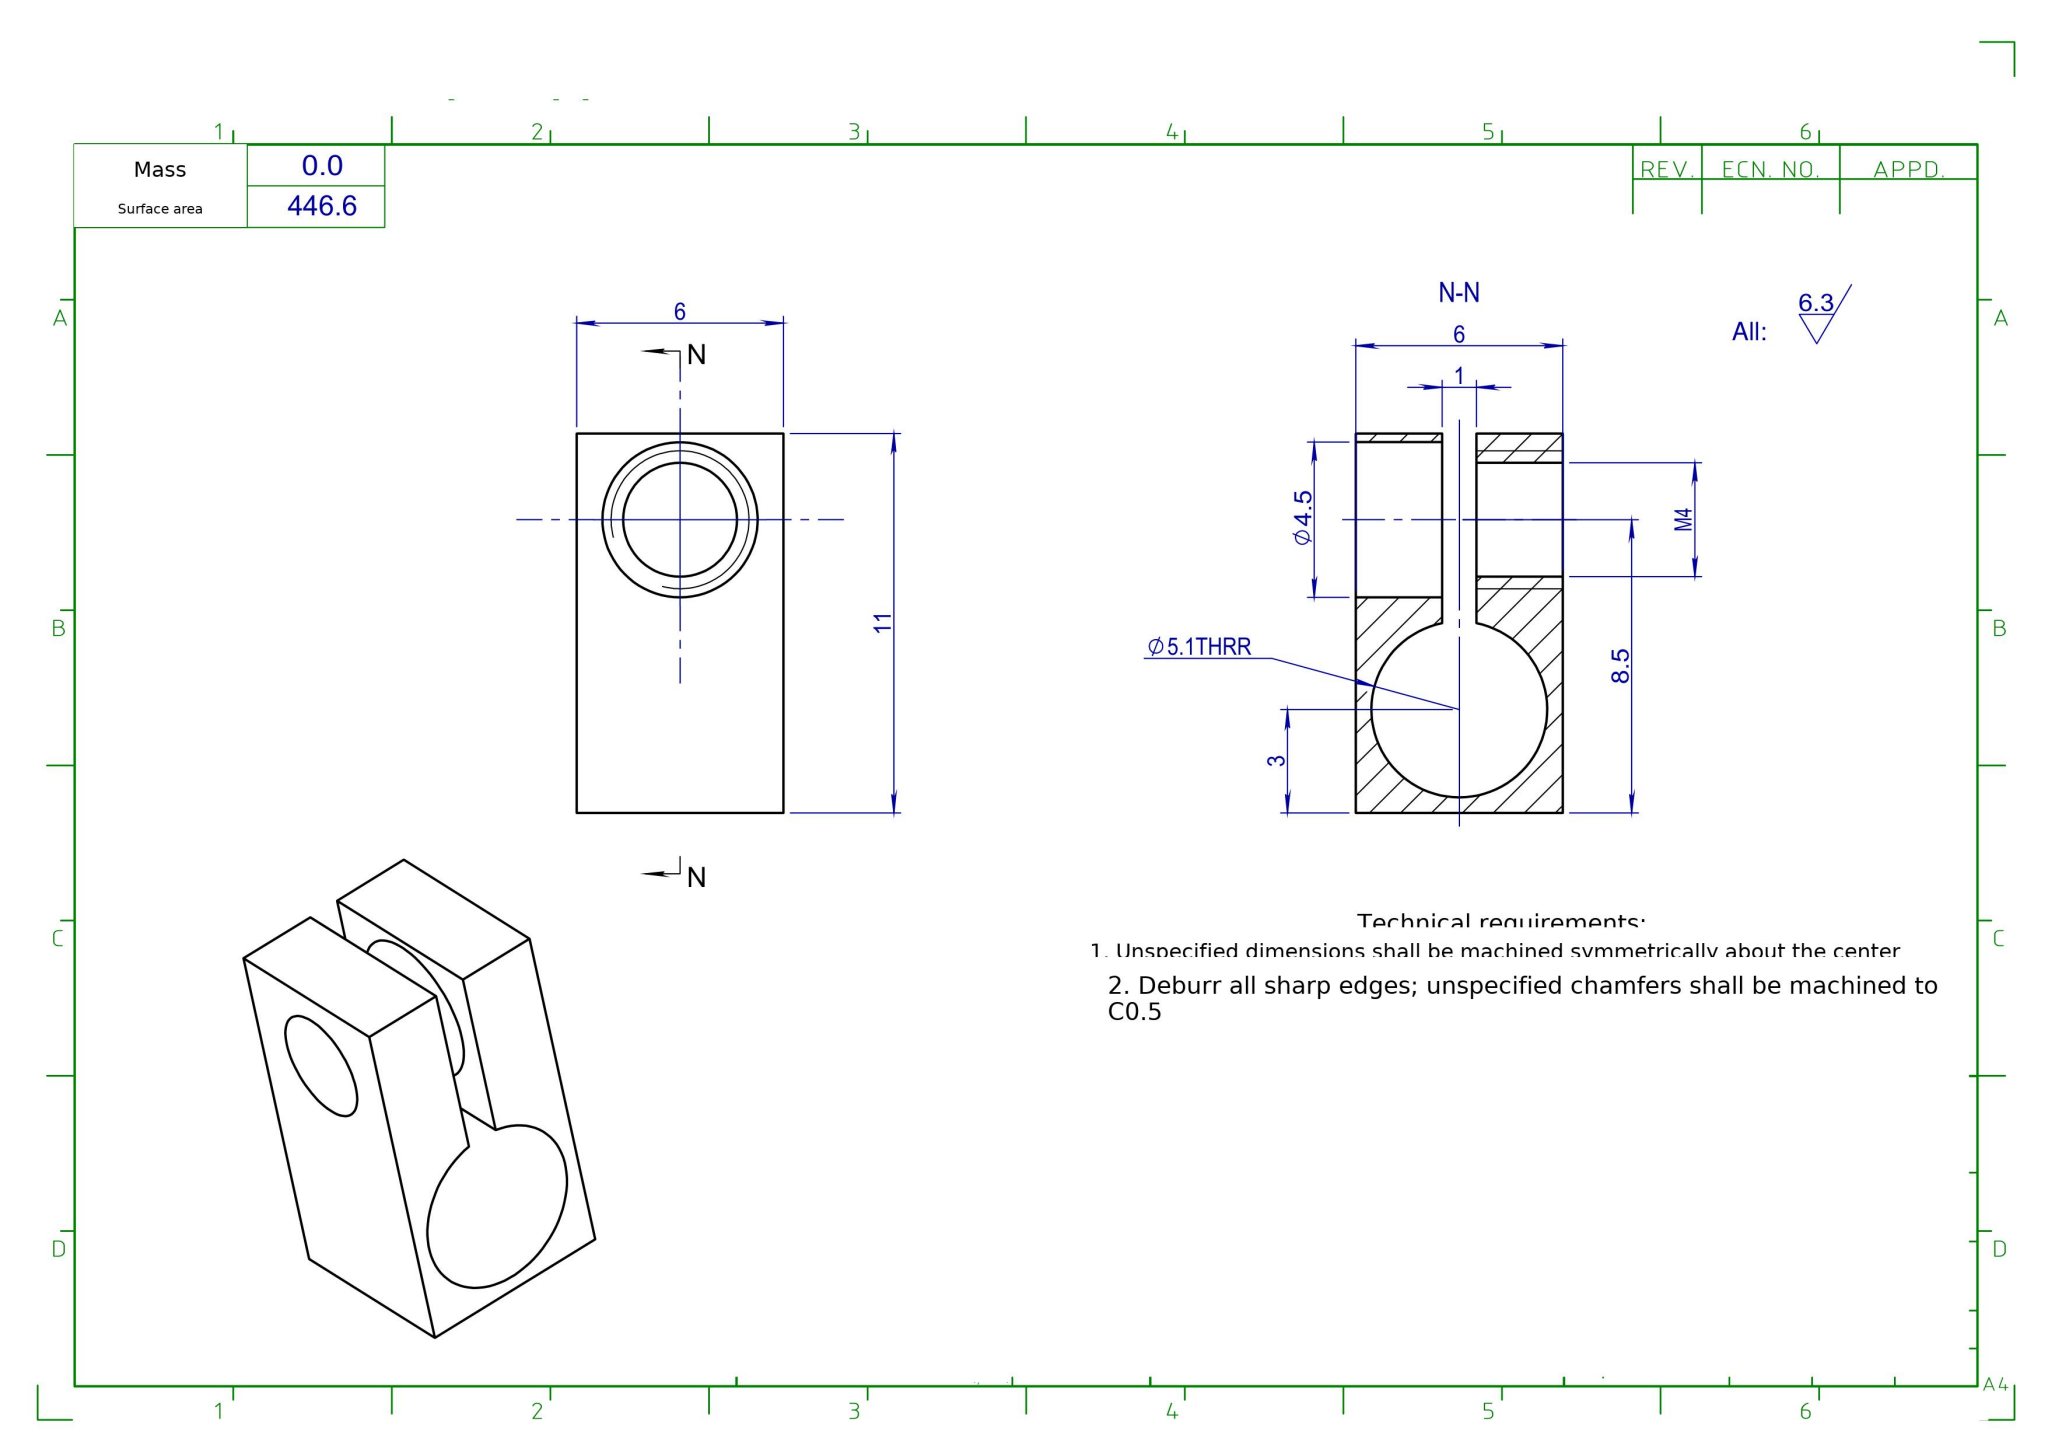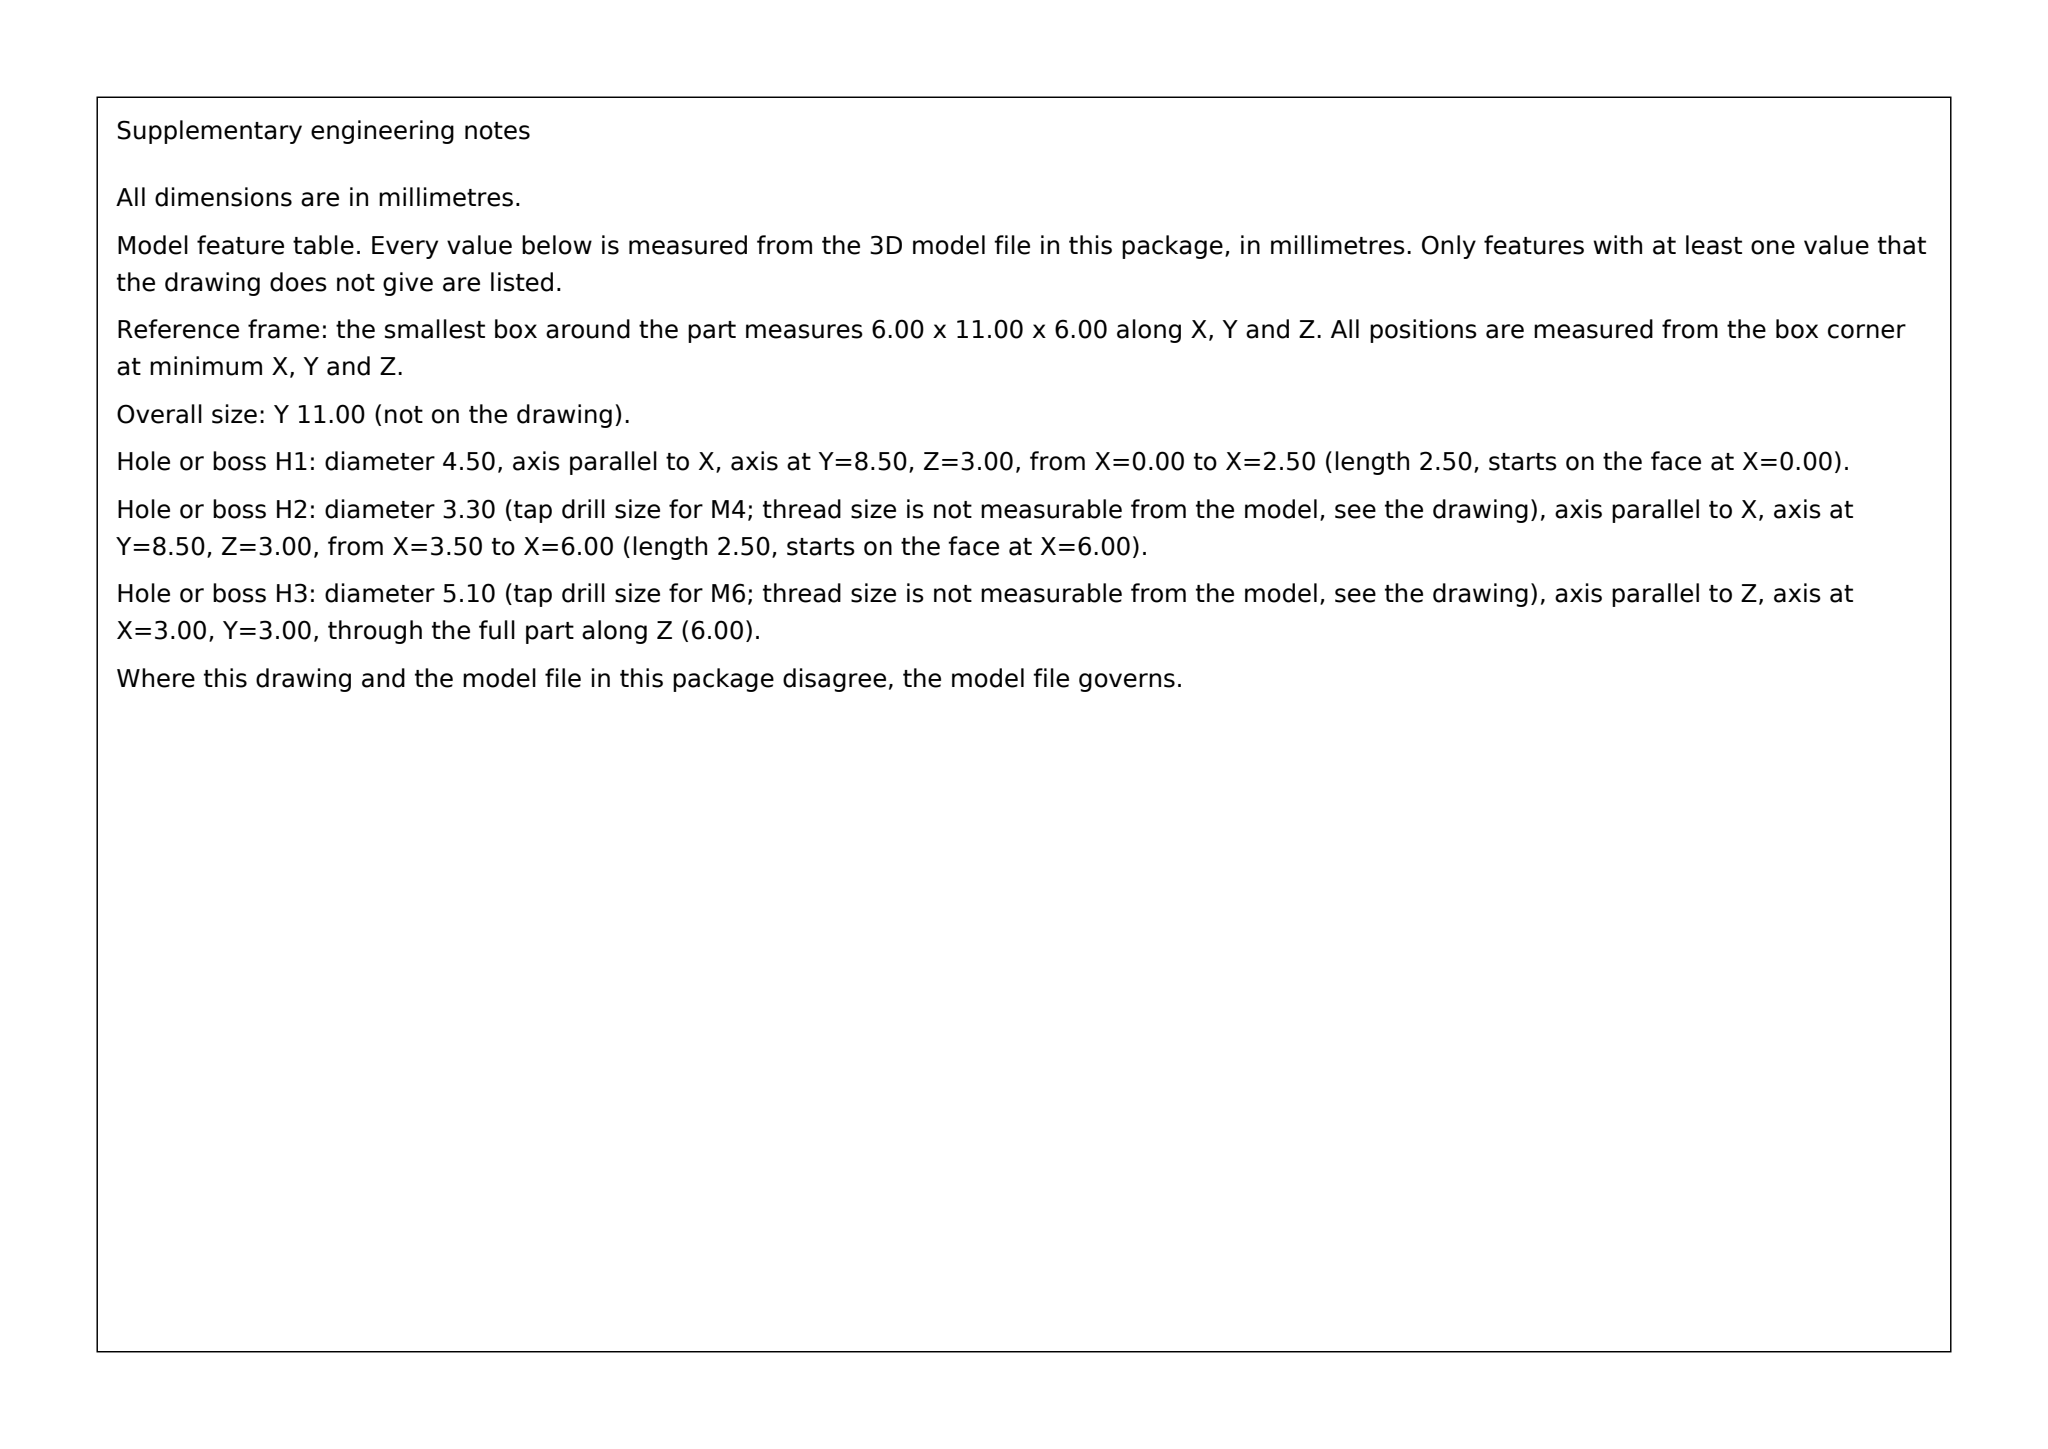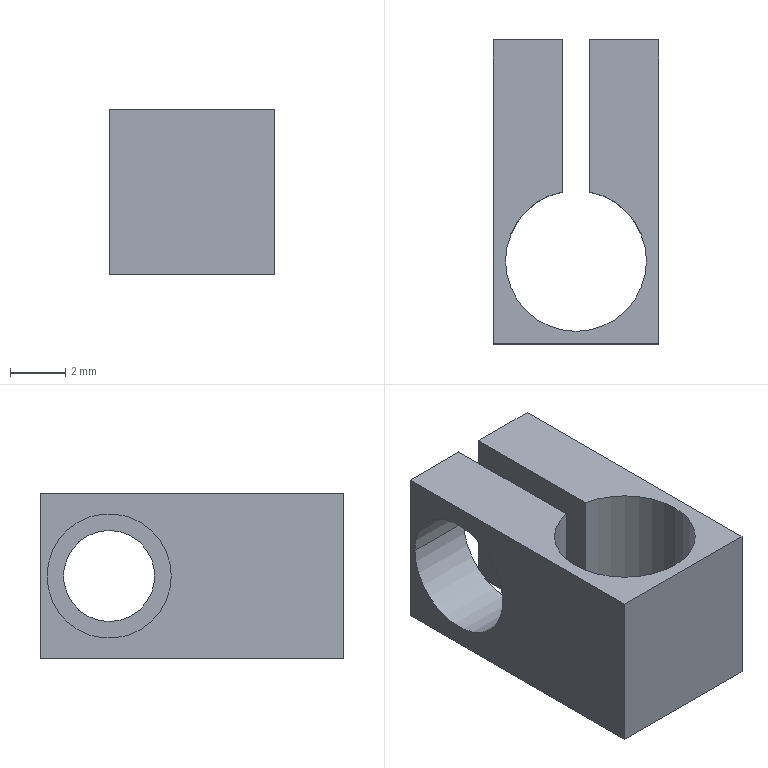Part | SolidWorks | mm | 1 solid | 16 faces | box 6 x 11 x 6 mm | volume 179 mm3 | plane 9 | cylinder 7 | commonest cylinder face diameters 5.1 x3 3.3 x2 4.5 x2
build123d program:
from build123d import *

# Parameters (mm, degrees)
SKETCH1_W             = 6
SKETCH1_H             = 11
EXTRUDE1_DEPTH        = 6
SKETCH2_R             = 2.55
CUT_EXTRUDE1_DEPTH    = 32.386
SKETCH4_W             = 1
SKETCH4_H             = 8
CUT_EXTRUDE3_DEPTH    = 32.386
SKETCH6_R             = 2.25
CUT_EXTRUDE5_DEPTH    = 2.5
M4_TAPPED_HOLE1_D     = 3.3
M4_TAPPED_HOLE1_DEPTH = 10.1
M4_TAPPED_HOLE1_TIP   = 0.9914


with BuildPart() as part:
    # Sketch1 → Extrude1 (new body)
    with BuildSketch(Plane.XY):
        with Locations((-13.52, -20.503)):
            Rectangle(SKETCH1_W, SKETCH1_H)
    extrude(amount=EXTRUDE1_DEPTH)

    # Sketch2 → Cut-Extrude1 (cut, through all)
    with BuildSketch(Plane.XY.offset(6)):
        with Locations((-13.52, -23.003)):
            Circle(SKETCH2_R)
    extrude(amount=-CUT_EXTRUDE1_DEPTH, mode=Mode.SUBTRACT)

    # Sketch4 → Cut-Extrude3 (cut, through all)
    with BuildSketch(Plane.XY.offset(6)):
        with Locations((-13.52, -19.003)):
            Rectangle(SKETCH4_W, SKETCH4_H)
    extrude(amount=-CUT_EXTRUDE3_DEPTH, mode=Mode.SUBTRACT)

    # Sketch6 → Cut-Extrude5 (cut)
    with BuildSketch(Plane.ZY.offset(16.52)):
        with Locations(Location((3, -17.503, 0), (0, 0, 270))):
            Circle(SKETCH6_R)
    extrude(amount=-CUT_EXTRUDE5_DEPTH, mode=Mode.SUBTRACT)

    # M4 Tapped Hole1
    with Locations(Plane.ZY.offset(13.02)):
        with Locations((3, -17.503)):
            Hole(M4_TAPPED_HOLE1_D / 2, depth=M4_TAPPED_HOLE1_DEPTH)
            with Locations((0, 0, -(M4_TAPPED_HOLE1_DEPTH + M4_TAPPED_HOLE1_TIP / 2))):  # 118° drill point
                Cone(0, M4_TAPPED_HOLE1_D / 2, M4_TAPPED_HOLE1_TIP, mode=Mode.SUBTRACT)


solid = part.part
STEP:
#1=CARTESIAN_POINT('',(-10.52,-17.503,1.35));
#2=VERTEX_POINT('',#1);
#3=CARTESIAN_POINT('',(-10.52,-17.503,4.65));
#4=VERTEX_POINT('',#3);
#5=CARTESIAN_POINT('',(-10.52,-17.503,3.));
#6=DIRECTION('',(-1.,-0.,0.));
#7=DIRECTION('',(0.,-1.,0.));
#8=AXIS2_PLACEMENT_3D('',#5,#6,#7);
#9=CIRCLE('',#8,1.65);
#10=EDGE_CURVE('',#2,#4,#9,.T.);
#11=ORIENTED_EDGE('',*,*,#10,.F.);
#12=CARTESIAN_POINT('',(-13.02,-17.503,1.35));
#13=VERTEX_POINT('',#12);
#14=CARTESIAN_POINT('',(-13.02,-17.503,1.35));
#15=DIRECTION('',(-1.,0.,0.));
#16=VECTOR('',#15,1000.);
#17=LINE('',#14,#16);
#18=EDGE_CURVE('',#2,#13,#17,.T.);
#19=ORIENTED_EDGE('',*,*,#18,.T.);
#20=CARTESIAN_POINT('',(-13.02,-17.503,4.65));
#21=VERTEX_POINT('',#20);
#22=CARTESIAN_POINT('',(-13.02,-17.503,3.));
#23=DIRECTION('',(-1.,0.,0.));
#24=DIRECTION('',(0.,0.,1.));
#25=AXIS2_PLACEMENT_3D('',#22,#23,#24);
#26=CIRCLE('',#25,1.65);
#27=EDGE_CURVE('',#13,#21,#26,.T.);
#28=ORIENTED_EDGE('',*,*,#27,.T.);
#29=CARTESIAN_POINT('',(-13.02,-17.503,4.65));
#30=DIRECTION('',(-1.,0.,0.));
#31=VECTOR('',#30,1000.);
#32=LINE('',#29,#31);
#33=EDGE_CURVE('',#4,#21,#32,.T.);
#34=ORIENTED_EDGE('',*,*,#33,.F.);
#35=EDGE_LOOP('',(#11,#19,#28,#34));
#36=FACE_OUTER_BOUND('',#35,.T.);
#37=CARTESIAN_POINT('',(-13.02,-17.503,3.));
#38=DIRECTION('',(-1.,0.,0.));
#39=DIRECTION('',(0.,0.,1.));
#40=AXIS2_PLACEMENT_3D('',#37,#38,#39);
#41=CYLINDRICAL_SURFACE('',#40,1.65);
#42=ADVANCED_FACE('',(#36),#41,.F.);
#43=CARTESIAN_POINT('',(-14.02,-15.253,3.));
#44=VERTEX_POINT('',#43);
#45=CARTESIAN_POINT('',(-14.02,-19.753,3.));
#46=VERTEX_POINT('',#45);
#47=CARTESIAN_POINT('',(-14.02,-17.503,3.));
#48=DIRECTION('',(-1.,-0.,0.));
#49=DIRECTION('',(0.,-1.,0.));
#50=AXIS2_PLACEMENT_3D('',#47,#48,#49);
#51=CIRCLE('',#50,2.25);
#52=EDGE_CURVE('',#44,#46,#51,.T.);
#53=ORIENTED_EDGE('',*,*,#52,.F.);
#54=CARTESIAN_POINT('',(-16.52,-15.253,3.));
#55=VERTEX_POINT('',#54);
#56=CARTESIAN_POINT('',(-14.02,-15.253,3.));
#57=DIRECTION('',(-1.,-0.,0.));
#58=VECTOR('',#57,1000.);
#59=LINE('',#56,#58);
#60=EDGE_CURVE('',#44,#55,#59,.T.);
#61=ORIENTED_EDGE('',*,*,#60,.T.);
#62=CARTESIAN_POINT('',(-16.52,-19.753,3.));
#63=VERTEX_POINT('',#62);
#64=CARTESIAN_POINT('',(-16.52,-17.503,3.));
#65=DIRECTION('',(-1.,-0.,0.));
#66=DIRECTION('',(0.,-1.,0.));
#67=AXIS2_PLACEMENT_3D('',#64,#65,#66);
#68=CIRCLE('',#67,2.25);
#69=EDGE_CURVE('',#55,#63,#68,.T.);
#70=ORIENTED_EDGE('',*,*,#69,.T.);
#71=CARTESIAN_POINT('',(-14.02,-19.753,3.));
#72=DIRECTION('',(-1.,-0.,0.));
#73=VECTOR('',#72,1000.);
#74=LINE('',#71,#73);
#75=EDGE_CURVE('',#46,#63,#74,.T.);
#76=ORIENTED_EDGE('',*,*,#75,.F.);
#77=EDGE_LOOP('',(#53,#61,#70,#76));
#78=FACE_OUTER_BOUND('',#77,.T.);
#79=CARTESIAN_POINT('',(-14.02,-17.503,3.));
#80=DIRECTION('',(-1.,-0.,0.));
#81=DIRECTION('',(0.,-1.,0.));
#82=AXIS2_PLACEMENT_3D('',#79,#80,#81);
#83=CYLINDRICAL_SURFACE('',#82,2.25);
#84=ADVANCED_FACE('',(#78),#83,.F.);
#85=CARTESIAN_POINT('',(-16.07,-23.003,0.));
#86=VERTEX_POINT('',#85);
#87=CARTESIAN_POINT('',(-10.97,-23.003,0.));
#88=VERTEX_POINT('',#87);
#89=CARTESIAN_POINT('',(-13.52,-23.003,0.));
#90=DIRECTION('',(0.,0.,1.));
#91=DIRECTION('',(1.,0.,0.));
#92=AXIS2_PLACEMENT_3D('',#89,#90,#91);
#93=CIRCLE('',#92,2.55);
#94=EDGE_CURVE('',#86,#88,#93,.T.);
#95=ORIENTED_EDGE('',*,*,#94,.F.);
#96=CARTESIAN_POINT('',(-16.07,-23.003,6.));
#97=VERTEX_POINT('',#96);
#98=CARTESIAN_POINT('',(-16.07,-23.003,0.));
#99=DIRECTION('',(0.,0.,1.));
#100=VECTOR('',#99,1000.);
#101=LINE('',#98,#100);
#102=EDGE_CURVE('',#86,#97,#101,.T.);
#103=ORIENTED_EDGE('',*,*,#102,.T.);
#104=CARTESIAN_POINT('',(-10.97,-23.003,6.));
#105=VERTEX_POINT('',#104);
#106=CARTESIAN_POINT('',(-13.52,-23.003,6.));
#107=DIRECTION('',(0.,0.,1.));
#108=DIRECTION('',(1.,0.,0.));
#109=AXIS2_PLACEMENT_3D('',#106,#107,#108);
#110=CIRCLE('',#109,2.55);
#111=EDGE_CURVE('',#97,#105,#110,.T.);
#112=ORIENTED_EDGE('',*,*,#111,.T.);
#113=CARTESIAN_POINT('',(-10.97,-23.003,0.));
#114=DIRECTION('',(0.,0.,1.));
#115=VECTOR('',#114,1000.);
#116=LINE('',#113,#115);
#117=EDGE_CURVE('',#88,#105,#116,.T.);
#118=ORIENTED_EDGE('',*,*,#117,.F.);
#119=EDGE_LOOP('',(#95,#103,#112,#118));
#120=FACE_OUTER_BOUND('',#119,.T.);
#121=CARTESIAN_POINT('',(-13.52,-23.003,0.));
#122=DIRECTION('',(0.,0.,1.));
#123=DIRECTION('',(1.,0.,0.));
#124=AXIS2_PLACEMENT_3D('',#121,#122,#123);
#125=CYLINDRICAL_SURFACE('',#124,2.55);
#126=ADVANCED_FACE('',(#120),#125,.F.);
#127=CARTESIAN_POINT('',(-13.02,-20.502,0.));
#128=VERTEX_POINT('',#127);
#129=CARTESIAN_POINT('',(-13.52,-23.003,0.));
#130=DIRECTION('',(0.,0.,1.));
#131=DIRECTION('',(1.,0.,0.));
#132=AXIS2_PLACEMENT_3D('',#129,#130,#131);
#133=CIRCLE('',#132,2.55);
#134=EDGE_CURVE('',#88,#128,#133,.T.);
#135=ORIENTED_EDGE('',*,*,#134,.F.);
#136=ORIENTED_EDGE('',*,*,#117,.T.);
#137=CARTESIAN_POINT('',(-13.02,-20.502,6.));
#138=VERTEX_POINT('',#137);
#139=CARTESIAN_POINT('',(-13.52,-23.003,6.));
#140=DIRECTION('',(0.,0.,1.));
#141=DIRECTION('',(1.,0.,0.));
#142=AXIS2_PLACEMENT_3D('',#139,#140,#141);
#143=CIRCLE('',#142,2.55);
#144=EDGE_CURVE('',#105,#138,#143,.T.);
#145=ORIENTED_EDGE('',*,*,#144,.T.);
#146=CARTESIAN_POINT('',(-13.02,-20.502,0.));
#147=DIRECTION('',(0.,0.,-1.));
#148=VECTOR('',#147,1000.);
#149=LINE('',#146,#148);
#150=EDGE_CURVE('',#138,#128,#149,.T.);
#151=ORIENTED_EDGE('',*,*,#150,.T.);
#152=EDGE_LOOP('',(#135,#136,#145,#151));
#153=FACE_OUTER_BOUND('',#152,.T.);
#154=CARTESIAN_POINT('',(-13.52,-23.003,0.));
#155=DIRECTION('',(0.,0.,1.));
#156=DIRECTION('',(1.,0.,0.));
#157=AXIS2_PLACEMENT_3D('',#154,#155,#156);
#158=CYLINDRICAL_SURFACE('',#157,2.55);
#159=ADVANCED_FACE('',(#153),#158,.F.);
#160=CARTESIAN_POINT('',(-14.02,-15.003,6.));
#161=VERTEX_POINT('',#160);
#162=CARTESIAN_POINT('',(-16.52,-15.003,6.));
#163=VERTEX_POINT('',#162);
#164=CARTESIAN_POINT('',(-16.52,-15.003,6.));
#165=DIRECTION('',(-1.,0.,0.));
#166=VECTOR('',#165,1000.);
#167=LINE('',#164,#166);
#168=EDGE_CURVE('',#161,#163,#167,.T.);
#169=ORIENTED_EDGE('',*,*,#168,.F.);
#170=CARTESIAN_POINT('',(-14.02,-15.003,0.));
#171=VERTEX_POINT('',#170);
#172=CARTESIAN_POINT('',(-14.02,-15.003,0.));
#173=DIRECTION('',(0.,0.,1.));
#174=VECTOR('',#173,1000.);
#175=LINE('',#172,#174);
#176=EDGE_CURVE('',#171,#161,#175,.T.);
#177=ORIENTED_EDGE('',*,*,#176,.F.);
#178=CARTESIAN_POINT('',(-16.52,-15.003,0.));
#179=VERTEX_POINT('',#178);
#180=CARTESIAN_POINT('',(-16.52,-15.003,0.));
#181=DIRECTION('',(-1.,0.,0.));
#182=VECTOR('',#181,1000.);
#183=LINE('',#180,#182);
#184=EDGE_CURVE('',#171,#179,#183,.T.);
#185=ORIENTED_EDGE('',*,*,#184,.T.);
#186=CARTESIAN_POINT('',(-16.52,-15.003,6.));
#187=DIRECTION('',(0.,0.,-1.));
#188=VECTOR('',#187,1000.);
#189=LINE('',#186,#188);
#190=EDGE_CURVE('',#163,#179,#189,.T.);
#191=ORIENTED_EDGE('',*,*,#190,.F.);
#192=EDGE_LOOP('',(#169,#177,#185,#191));
#193=FACE_OUTER_BOUND('',#192,.T.);
#194=CARTESIAN_POINT('',(-16.52,-15.003,6.));
#195=DIRECTION('',(0.,-1.,0.));
#196=DIRECTION('',(0.,0.,-1.));
#197=AXIS2_PLACEMENT_3D('',#194,#195,#196);
#198=PLANE('',#197);
#199=ADVANCED_FACE('',(#193),#198,.F.);
#200=CARTESIAN_POINT('',(-16.52,-17.503,3.));
#201=DIRECTION('',(-1.,-0.,0.));
#202=DIRECTION('',(0.,-1.,0.));
#203=AXIS2_PLACEMENT_3D('',#200,#201,#202);
#204=CIRCLE('',#203,2.25);
#205=EDGE_CURVE('',#63,#55,#204,.T.);
#206=ORIENTED_EDGE('',*,*,#205,.F.);
#207=ORIENTED_EDGE('',*,*,#69,.F.);
#208=EDGE_LOOP('',(#206,#207));
#209=FACE_BOUND('',#208,.T.);
#210=CARTESIAN_POINT('',(-16.52,-26.003,0.));
#211=VERTEX_POINT('',#210);
#212=CARTESIAN_POINT('',(-16.52,-15.003,0.));
#213=DIRECTION('',(0.,-1.,0.));
#214=VECTOR('',#213,1000.);
#215=LINE('',#212,#214);
#216=EDGE_CURVE('',#179,#211,#215,.T.);
#217=ORIENTED_EDGE('',*,*,#216,.T.);
#218=CARTESIAN_POINT('',(-16.52,-26.003,6.));
#219=VERTEX_POINT('',#218);
#220=CARTESIAN_POINT('',(-16.52,-26.003,6.));
#221=DIRECTION('',(0.,0.,-1.));
#222=VECTOR('',#221,1000.);
#223=LINE('',#220,#222);
#224=EDGE_CURVE('',#219,#211,#223,.T.);
#225=ORIENTED_EDGE('',*,*,#224,.F.);
#226=CARTESIAN_POINT('',(-16.52,-15.003,6.));
#227=DIRECTION('',(0.,-1.,0.));
#228=VECTOR('',#227,1000.);
#229=LINE('',#226,#228);
#230=EDGE_CURVE('',#163,#219,#229,.T.);
#231=ORIENTED_EDGE('',*,*,#230,.F.);
#232=ORIENTED_EDGE('',*,*,#190,.T.);
#233=EDGE_LOOP('',(#217,#225,#231,#232));
#234=FACE_OUTER_BOUND('',#233,.T.);
#235=CARTESIAN_POINT('',(-16.52,-15.003,6.));
#236=DIRECTION('',(1.,0.,0.));
#237=DIRECTION('',(0.,0.,-1.));
#238=AXIS2_PLACEMENT_3D('',#235,#236,#237);
#239=PLANE('',#238);
#240=ADVANCED_FACE('',(#209,#234),#239,.F.);
#241=CARTESIAN_POINT('',(-10.52,-26.003,0.));
#242=VERTEX_POINT('',#241);
#243=CARTESIAN_POINT('',(-16.52,-26.003,0.));
#244=DIRECTION('',(1.,0.,0.));
#245=VECTOR('',#244,1000.);
#246=LINE('',#243,#245);
#247=EDGE_CURVE('',#211,#242,#246,.T.);
#248=ORIENTED_EDGE('',*,*,#247,.T.);
#249=CARTESIAN_POINT('',(-10.52,-26.003,6.));
#250=VERTEX_POINT('',#249);
#251=CARTESIAN_POINT('',(-10.52,-26.003,6.));
#252=DIRECTION('',(0.,0.,-1.));
#253=VECTOR('',#252,1000.);
#254=LINE('',#251,#253);
#255=EDGE_CURVE('',#250,#242,#254,.T.);
#256=ORIENTED_EDGE('',*,*,#255,.F.);
#257=CARTESIAN_POINT('',(-16.52,-26.003,6.));
#258=DIRECTION('',(1.,0.,0.));
#259=VECTOR('',#258,1000.);
#260=LINE('',#257,#259);
#261=EDGE_CURVE('',#219,#250,#260,.T.);
#262=ORIENTED_EDGE('',*,*,#261,.F.);
#263=ORIENTED_EDGE('',*,*,#224,.T.);
#264=EDGE_LOOP('',(#248,#256,#262,#263));
#265=FACE_OUTER_BOUND('',#264,.T.);
#266=CARTESIAN_POINT('',(-16.52,-26.003,6.));
#267=DIRECTION('',(0.,1.,0.));
#268=DIRECTION('',(0.,0.,1.));
#269=AXIS2_PLACEMENT_3D('',#266,#267,#268);
#270=PLANE('',#269);
#271=ADVANCED_FACE('',(#265),#270,.F.);
#272=CARTESIAN_POINT('',(-10.52,-17.503,3.));
#273=DIRECTION('',(-1.,-0.,0.));
#274=DIRECTION('',(0.,-1.,0.));
#275=AXIS2_PLACEMENT_3D('',#272,#273,#274);
#276=CIRCLE('',#275,1.65);
#277=EDGE_CURVE('',#4,#2,#276,.T.);
#278=ORIENTED_EDGE('',*,*,#277,.T.);
#279=ORIENTED_EDGE('',*,*,#10,.T.);
#280=EDGE_LOOP('',(#278,#279));
#281=FACE_BOUND('',#280,.T.);
#282=CARTESIAN_POINT('',(-10.52,-15.003,0.));
#283=VERTEX_POINT('',#282);
#284=CARTESIAN_POINT('',(-10.52,-15.003,0.));
#285=DIRECTION('',(-0.,1.,0.));
#286=VECTOR('',#285,1000.);
#287=LINE('',#284,#286);
#288=EDGE_CURVE('',#242,#283,#287,.T.);
#289=ORIENTED_EDGE('',*,*,#288,.T.);
#290=CARTESIAN_POINT('',(-10.52,-15.003,6.));
#291=VERTEX_POINT('',#290);
#292=CARTESIAN_POINT('',(-10.52,-15.003,6.));
#293=DIRECTION('',(0.,0.,-1.));
#294=VECTOR('',#293,1000.);
#295=LINE('',#292,#294);
#296=EDGE_CURVE('',#291,#283,#295,.T.);
#297=ORIENTED_EDGE('',*,*,#296,.F.);
#298=CARTESIAN_POINT('',(-10.52,-15.003,6.));
#299=DIRECTION('',(-0.,1.,0.));
#300=VECTOR('',#299,1000.);
#301=LINE('',#298,#300);
#302=EDGE_CURVE('',#250,#291,#301,.T.);
#303=ORIENTED_EDGE('',*,*,#302,.F.);
#304=ORIENTED_EDGE('',*,*,#255,.T.);
#305=EDGE_LOOP('',(#289,#297,#303,#304));
#306=FACE_OUTER_BOUND('',#305,.T.);
#307=CARTESIAN_POINT('',(-10.52,-15.003,6.));
#308=DIRECTION('',(-1.,-0.,0.));
#309=DIRECTION('',(0.,-1.,0.));
#310=AXIS2_PLACEMENT_3D('',#307,#308,#309);
#311=PLANE('',#310);
#312=ADVANCED_FACE('',(#281,#306),#311,.F.);
#313=CARTESIAN_POINT('',(-13.02,-15.003,0.));
#314=VERTEX_POINT('',#313);
#315=CARTESIAN_POINT('',(-16.52,-15.003,0.));
#316=DIRECTION('',(-1.,0.,0.));
#317=VECTOR('',#316,1000.);
#318=LINE('',#315,#317);
#319=EDGE_CURVE('',#283,#314,#318,.T.);
#320=ORIENTED_EDGE('',*,*,#319,.T.);
#321=CARTESIAN_POINT('',(-13.02,-15.003,6.));
#322=VERTEX_POINT('',#321);
#323=CARTESIAN_POINT('',(-13.02,-15.003,0.));
#324=DIRECTION('',(0.,0.,1.));
#325=VECTOR('',#324,1000.);
#326=LINE('',#323,#325);
#327=EDGE_CURVE('',#314,#322,#326,.T.);
#328=ORIENTED_EDGE('',*,*,#327,.T.);
#329=CARTESIAN_POINT('',(-16.52,-15.003,6.));
#330=DIRECTION('',(-1.,0.,0.));
#331=VECTOR('',#330,1000.);
#332=LINE('',#329,#331);
#333=EDGE_CURVE('',#291,#322,#332,.T.);
#334=ORIENTED_EDGE('',*,*,#333,.F.);
#335=ORIENTED_EDGE('',*,*,#296,.T.);
#336=EDGE_LOOP('',(#320,#328,#334,#335));
#337=FACE_OUTER_BOUND('',#336,.T.);
#338=CARTESIAN_POINT('',(-16.52,-15.003,6.));
#339=DIRECTION('',(0.,-1.,0.));
#340=DIRECTION('',(0.,0.,-1.));
#341=AXIS2_PLACEMENT_3D('',#338,#339,#340);
#342=PLANE('',#341);
#343=ADVANCED_FACE('',(#337),#342,.F.);
#344=CARTESIAN_POINT('',(-14.02,-20.502,6.));
#345=VERTEX_POINT('',#344);
#346=CARTESIAN_POINT('',(-14.02,-15.003,6.));
#347=DIRECTION('',(0.,-1.,0.));
#348=VECTOR('',#347,1000.);
#349=LINE('',#346,#348);
#350=EDGE_CURVE('',#161,#345,#349,.T.);
#351=ORIENTED_EDGE('',*,*,#350,.F.);
#352=ORIENTED_EDGE('',*,*,#168,.T.);
#353=ORIENTED_EDGE('',*,*,#230,.T.);
#354=ORIENTED_EDGE('',*,*,#261,.T.);
#355=ORIENTED_EDGE('',*,*,#302,.T.);
#356=ORIENTED_EDGE('',*,*,#333,.T.);
#357=CARTESIAN_POINT('',(-13.02,-15.003,6.));
#358=DIRECTION('',(0.,1.,0.));
#359=VECTOR('',#358,1000.);
#360=LINE('',#357,#359);
#361=EDGE_CURVE('',#138,#322,#360,.T.);
#362=ORIENTED_EDGE('',*,*,#361,.F.);
#363=ORIENTED_EDGE('',*,*,#144,.F.);
#364=ORIENTED_EDGE('',*,*,#111,.F.);
#365=CARTESIAN_POINT('',(-13.52,-23.003,6.));
#366=DIRECTION('',(0.,0.,1.));
#367=DIRECTION('',(1.,0.,0.));
#368=AXIS2_PLACEMENT_3D('',#365,#366,#367);
#369=CIRCLE('',#368,2.55);
#370=EDGE_CURVE('',#345,#97,#369,.T.);
#371=ORIENTED_EDGE('',*,*,#370,.F.);
#372=EDGE_LOOP('',(#351,#352,#353,#354,#355,#356,#362,#363,#364,#371));
#373=FACE_OUTER_BOUND('',#372,.T.);
#374=CARTESIAN_POINT('',(-16.52,-26.003,6.));
#375=DIRECTION('',(0.,0.,1.));
#376=DIRECTION('',(1.,0.,0.));
#377=AXIS2_PLACEMENT_3D('',#374,#375,#376);
#378=PLANE('',#377);
#379=ADVANCED_FACE('',(#373),#378,.T.);
#380=ORIENTED_EDGE('',*,*,#184,.F.);
#381=CARTESIAN_POINT('',(-14.02,-20.502,0.));
#382=VERTEX_POINT('',#381);
#383=CARTESIAN_POINT('',(-14.02,-15.003,0.));
#384=DIRECTION('',(0.,-1.,0.));
#385=VECTOR('',#384,1000.);
#386=LINE('',#383,#385);
#387=EDGE_CURVE('',#171,#382,#386,.T.);
#388=ORIENTED_EDGE('',*,*,#387,.T.);
#389=CARTESIAN_POINT('',(-13.52,-23.003,0.));
#390=DIRECTION('',(0.,0.,1.));
#391=DIRECTION('',(1.,0.,0.));
#392=AXIS2_PLACEMENT_3D('',#389,#390,#391);
#393=CIRCLE('',#392,2.55);
#394=EDGE_CURVE('',#382,#86,#393,.T.);
#395=ORIENTED_EDGE('',*,*,#394,.T.);
#396=ORIENTED_EDGE('',*,*,#94,.T.);
#397=ORIENTED_EDGE('',*,*,#134,.T.);
#398=CARTESIAN_POINT('',(-13.02,-15.003,0.));
#399=DIRECTION('',(0.,1.,0.));
#400=VECTOR('',#399,1000.);
#401=LINE('',#398,#400);
#402=EDGE_CURVE('',#128,#314,#401,.T.);
#403=ORIENTED_EDGE('',*,*,#402,.T.);
#404=ORIENTED_EDGE('',*,*,#319,.F.);
#405=ORIENTED_EDGE('',*,*,#288,.F.);
#406=ORIENTED_EDGE('',*,*,#247,.F.);
#407=ORIENTED_EDGE('',*,*,#216,.F.);
#408=EDGE_LOOP('',(#380,#388,#395,#396,#397,#403,#404,#405,#406,#407));
#409=FACE_OUTER_BOUND('',#408,.T.);
#410=CARTESIAN_POINT('',(-16.52,-26.003,0.));
#411=DIRECTION('',(0.,0.,1.));
#412=DIRECTION('',(1.,0.,0.));
#413=AXIS2_PLACEMENT_3D('',#410,#411,#412);
#414=PLANE('',#413);
#415=ADVANCED_FACE('',(#409),#414,.F.);
#416=ORIENTED_EDGE('',*,*,#102,.F.);
#417=ORIENTED_EDGE('',*,*,#394,.F.);
#418=CARTESIAN_POINT('',(-14.02,-20.502,0.));
#419=DIRECTION('',(0.,0.,1.));
#420=VECTOR('',#419,1000.);
#421=LINE('',#418,#420);
#422=EDGE_CURVE('',#382,#345,#421,.T.);
#423=ORIENTED_EDGE('',*,*,#422,.T.);
#424=ORIENTED_EDGE('',*,*,#370,.T.);
#425=EDGE_LOOP('',(#416,#417,#423,#424));
#426=FACE_OUTER_BOUND('',#425,.T.);
#427=CARTESIAN_POINT('',(-13.52,-23.003,0.));
#428=DIRECTION('',(0.,0.,1.));
#429=DIRECTION('',(1.,0.,0.));
#430=AXIS2_PLACEMENT_3D('',#427,#428,#429);
#431=CYLINDRICAL_SURFACE('',#430,2.55);
#432=ADVANCED_FACE('',(#426),#431,.F.);
#433=CARTESIAN_POINT('',(-13.02,-17.503,3.));
#434=DIRECTION('',(-1.,0.,0.));
#435=DIRECTION('',(0.,0.,1.));
#436=AXIS2_PLACEMENT_3D('',#433,#434,#435);
#437=CIRCLE('',#436,1.65);
#438=EDGE_CURVE('',#21,#13,#437,.T.);
#439=ORIENTED_EDGE('',*,*,#438,.F.);
#440=ORIENTED_EDGE('',*,*,#27,.F.);
#441=EDGE_LOOP('',(#439,#440));
#442=FACE_BOUND('',#441,.T.);
#443=ORIENTED_EDGE('',*,*,#361,.T.);
#444=ORIENTED_EDGE('',*,*,#327,.F.);
#445=ORIENTED_EDGE('',*,*,#402,.F.);
#446=ORIENTED_EDGE('',*,*,#150,.F.);
#447=EDGE_LOOP('',(#443,#444,#445,#446));
#448=FACE_OUTER_BOUND('',#447,.T.);
#449=CARTESIAN_POINT('',(-13.02,-15.003,0.));
#450=DIRECTION('',(1.,0.,0.));
#451=DIRECTION('',(0.,0.,-1.));
#452=AXIS2_PLACEMENT_3D('',#449,#450,#451);
#453=PLANE('',#452);
#454=ADVANCED_FACE('',(#442,#448),#453,.F.);
#455=CARTESIAN_POINT('',(-14.02,-17.503,3.));
#456=DIRECTION('',(-1.,-0.,0.));
#457=DIRECTION('',(0.,-1.,0.));
#458=AXIS2_PLACEMENT_3D('',#455,#456,#457);
#459=CIRCLE('',#458,2.25);
#460=EDGE_CURVE('',#46,#44,#459,.T.);
#461=ORIENTED_EDGE('',*,*,#460,.T.);
#462=ORIENTED_EDGE('',*,*,#52,.T.);
#463=EDGE_LOOP('',(#461,#462));
#464=FACE_BOUND('',#463,.T.);
#465=ORIENTED_EDGE('',*,*,#387,.F.);
#466=ORIENTED_EDGE('',*,*,#176,.T.);
#467=ORIENTED_EDGE('',*,*,#350,.T.);
#468=ORIENTED_EDGE('',*,*,#422,.F.);
#469=EDGE_LOOP('',(#465,#466,#467,#468));
#470=FACE_OUTER_BOUND('',#469,.T.);
#471=CARTESIAN_POINT('',(-14.02,-15.003,0.));
#472=DIRECTION('',(-1.,-0.,0.));
#473=DIRECTION('',(0.,-1.,0.));
#474=AXIS2_PLACEMENT_3D('',#471,#472,#473);
#475=PLANE('',#474);
#476=ADVANCED_FACE('',(#464,#470),#475,.F.);
#477=ORIENTED_EDGE('',*,*,#60,.F.);
#478=ORIENTED_EDGE('',*,*,#460,.F.);
#479=ORIENTED_EDGE('',*,*,#75,.T.);
#480=ORIENTED_EDGE('',*,*,#205,.T.);
#481=EDGE_LOOP('',(#477,#478,#479,#480));
#482=FACE_OUTER_BOUND('',#481,.T.);
#483=CARTESIAN_POINT('',(-14.02,-17.503,3.));
#484=DIRECTION('',(-1.,-0.,0.));
#485=DIRECTION('',(0.,-1.,0.));
#486=AXIS2_PLACEMENT_3D('',#483,#484,#485);
#487=CYLINDRICAL_SURFACE('',#486,2.25);
#488=ADVANCED_FACE('',(#482),#487,.F.);
#489=ORIENTED_EDGE('',*,*,#18,.F.);
#490=ORIENTED_EDGE('',*,*,#277,.F.);
#491=ORIENTED_EDGE('',*,*,#33,.T.);
#492=ORIENTED_EDGE('',*,*,#438,.T.);
#493=EDGE_LOOP('',(#489,#490,#491,#492));
#494=FACE_OUTER_BOUND('',#493,.T.);
#495=CARTESIAN_POINT('',(-13.02,-17.503,3.));
#496=DIRECTION('',(-1.,0.,0.));
#497=DIRECTION('',(0.,0.,1.));
#498=AXIS2_PLACEMENT_3D('',#495,#496,#497);
#499=CYLINDRICAL_SURFACE('',#498,1.65);
#500=ADVANCED_FACE('',(#494),#499,.F.);
#501=CLOSED_SHELL('',(#42,#84,#126,#159,#199,#240,#271,#312,#343,#379,#415,#432,#454,#476,#488,#500));
#502=MANIFOLD_SOLID_BREP('',#501);
#503=CARTESIAN_POINT('',(0.,0.,0.));
#504=DIRECTION('',(0.,0.,1.));
#505=DIRECTION('',(1.,0.,0.));
#506=AXIS2_PLACEMENT_3D('',#503,#504,#505);
#507=(LENGTH_UNIT()NAMED_UNIT(*)SI_UNIT(.MILLI.,.METRE.));
#508=UNCERTAINTY_MEASURE_WITH_UNIT(LENGTH_MEASURE(0.00001),#507,'','');
#509=(NAMED_UNIT(*)PLANE_ANGLE_UNIT()SI_UNIT($,.RADIAN.));
#510=(NAMED_UNIT(*)SI_UNIT($,.STERADIAN.)SOLID_ANGLE_UNIT());
#511=(GEOMETRIC_REPRESENTATION_CONTEXT(3)GLOBAL_UNCERTAINTY_ASSIGNED_CONTEXT((#508))GLOBAL_UNIT_ASSIGNED_CONTEXT((#507,#509,#510))REPRESENTATION_CONTEXT('',''));
#512=ADVANCED_BREP_SHAPE_REPRESENTATION('',(#502,#506),#511);